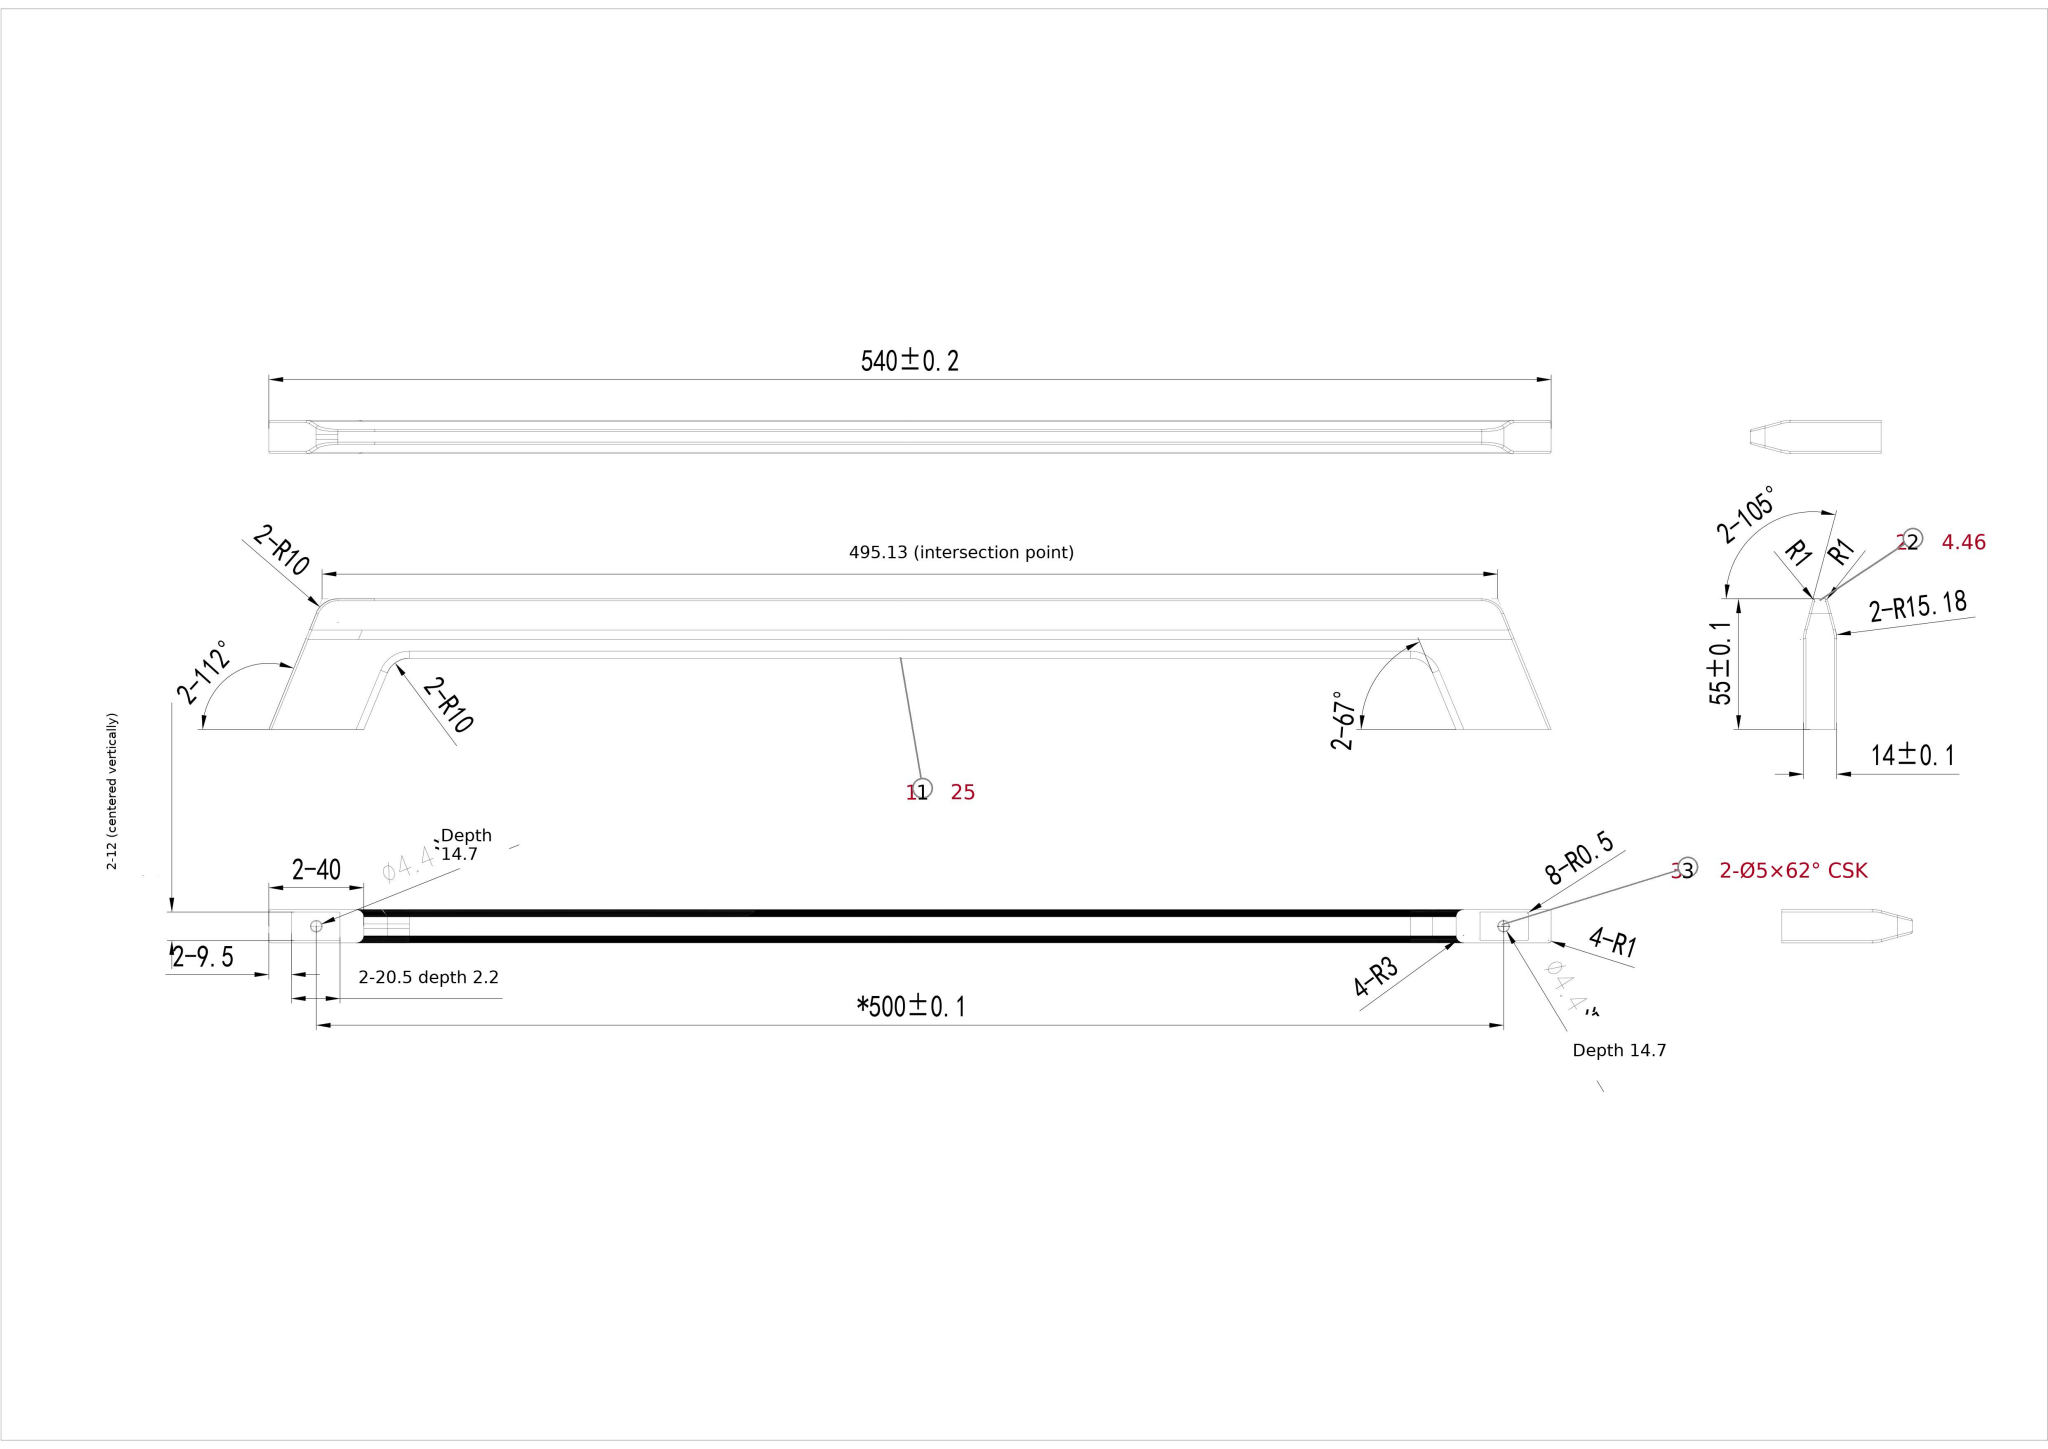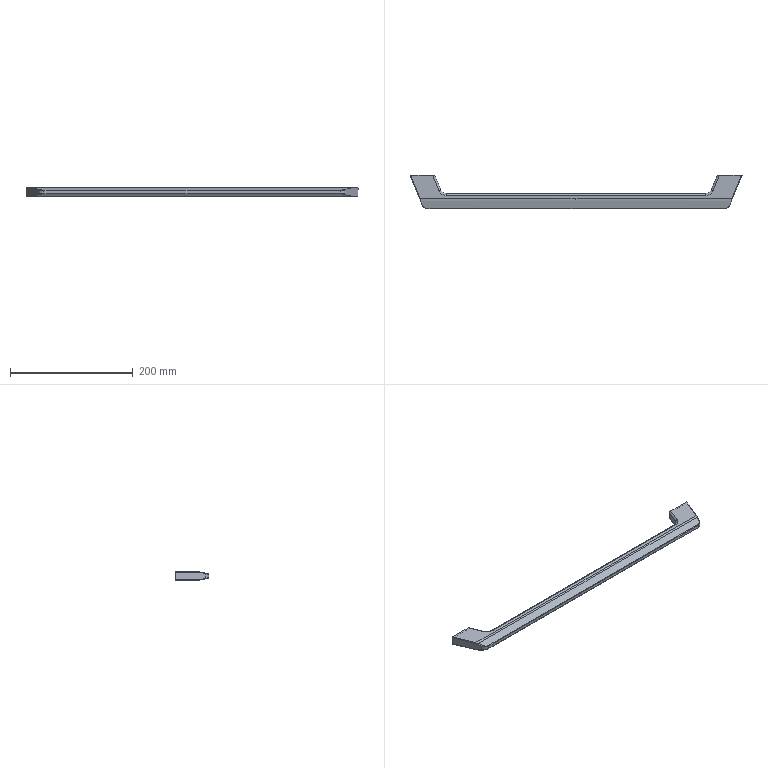Part | SolidWorks | mm | 1 solid | 81 faces | box 540 x 55 x 14 mm | volume 176996 mm3 | cylinder 41 | plane 24 | spline 12 | cone 4 | commonest cylinder face diameters 2 x14 1 x8 6 x6 30.387 x5 4.4 x4 20 x4